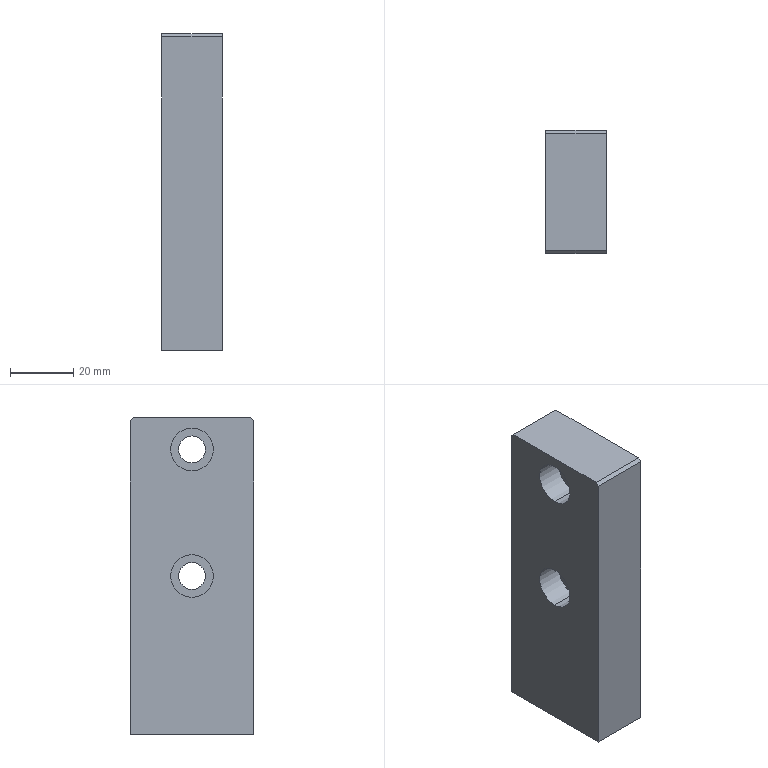Component | SolidWorks | TAR-02-017RightSupportPlate-1 | 1 solid | 26 faces | box 19 x 39 x 100 mm | volume 68972 mm3 | cylinder 12 | plane 10 | cone 4 | commonest cylinder face diameters 6.8 x4 13.5 x4 8.5 x4
build123d program:
from build123d import *

# Parameters (mm, degrees)
SKETCH1_W                                            = 100
SKETCH1_H                                            = 39
BOSS_EXTRUDE1_DEPTH                                  = 19
CYLINDRICAL_COUNTERSUNK_HOLE_FOR_M6_HEX_D            = 8.5
CYLINDRICAL_COUNTERSUNK_HOLE_FOR_M6_HEX_CBORE_D      = 13.5
CYLINDRICAL_COUNTERSUNK_HOLE_FOR_M6_HEX_CBORE_DEPTH  = 8.5
M6_HEX_HEAD_BOLT_CYLINDRICAL_COUNTERSUNK_D           = 8.5
M6_HEX_HEAD_BOLT_CYLINDRICAL_COUNTERSUNK_CBORE_D     = 13.5
M6_HEX_HEAD_BOLT_CYLINDRICAL_COUNTERSUNK_CBORE_DEPTH = 8.5
CHAMFER1_SIZE                                        = 1
M8_TAPPED_HOLE1_D                                    = 6.8
M8_TAPPED_HOLE1_DEPTH                                = 19.75
M8_TAPPED_HOLE1_TIP                                  = 2.043


with BuildPart() as part:
    # Sketch1 → Boss-Extrude1 (new body)
    with BuildSketch(Plane(origin=(0, 0, 0), x_dir=(0, 0, -1), z_dir=(1, 0, 0))):
        Rectangle(SKETCH1_W, SKETCH1_H)
    extrude(amount=BOSS_EXTRUDE1_DEPTH)

    # Cylindrical Countersunk Hole for M6 Hex (through all)
    with Locations(Plane(origin=(19, 0, 40), x_dir=(0, 0, 1), z_dir=(1, 0, 0))):
        with Locations((0, 0)):
            CounterBoreHole(CYLINDRICAL_COUNTERSUNK_HOLE_FOR_M6_HEX_D / 2, CYLINDRICAL_COUNTERSUNK_HOLE_FOR_M6_HEX_CBORE_D / 2, CYLINDRICAL_COUNTERSUNK_HOLE_FOR_M6_HEX_CBORE_DEPTH)

    # M6 Hex Head Bolt Cylindrical Countersunk (through all)
    with Locations(Plane(origin=(19, 0, 0), x_dir=(0, 0, 1), z_dir=(1, 0, 0))):
        with Locations((0, 0)):
            CounterBoreHole(M6_HEX_HEAD_BOLT_CYLINDRICAL_COUNTERSUNK_D / 2, M6_HEX_HEAD_BOLT_CYLINDRICAL_COUNTERSUNK_CBORE_D / 2, M6_HEX_HEAD_BOLT_CYLINDRICAL_COUNTERSUNK_CBORE_DEPTH)

    # Chamfer1
    chamfer1_edges = [part.edges().sort_by_distance(p)[0] for p in [
        (9.5, 19.5, 50),
        (9.5, -19.5, 50),
    ]]
    chamfer(chamfer1_edges, length=CHAMFER1_SIZE)

    # M8 Tapped Hole1
    with Locations(Plane(origin=(9.5, 10, -50), x_dir=(-1, 0, 0), z_dir=(0, 0, -1))):
        with Locations((0, 0), (0, -20)):
            Hole(M8_TAPPED_HOLE1_D / 2, depth=M8_TAPPED_HOLE1_DEPTH)
            with Locations((0, 0, -(M8_TAPPED_HOLE1_DEPTH + M8_TAPPED_HOLE1_TIP / 2))):  # 118° drill point
                Cone(0, M8_TAPPED_HOLE1_D / 2, M8_TAPPED_HOLE1_TIP, mode=Mode.SUBTRACT)


solid = part.part

# Placed as in the assembly
solid = solid.moved(Location((-44.891, 9.288, 59.5), (0, 0, 180)))
STEP:
#1=COLOUR_RGB('',0.7922,0.8196,0.9333);
#2=FILL_AREA_STYLE_COLOUR('',#1);
#3=FILL_AREA_STYLE('',(#2));
#4=SURFACE_STYLE_FILL_AREA(#3);
#5=SURFACE_SIDE_STYLE('',(#4));
#6=SURFACE_STYLE_USAGE(.BOTH.,#5);
#7=PRESENTATION_STYLE_ASSIGNMENT((#6));
#8=CARTESIAN_POINT('',(-2.275,-0.02804,1.152));
#9=VERTEX_POINT('',#8);
#10=CARTESIAN_POINT('',(-2.008,-0.02804,1.152));
#11=VERTEX_POINT('',#10);
#12=CARTESIAN_POINT('',(-2.141,-0.02804,1.152));
#13=DIRECTION('',(0.,0.,-1.));
#14=DIRECTION('',(1.,-0.,0.));
#15=AXIS2_PLACEMENT_3D('',#12,#13,#14);
#16=CIRCLE('',#15,0.1339);
#17=EDGE_CURVE('',#9,#11,#16,.T.);
#18=ORIENTED_EDGE('',*,*,#17,.F.);
#19=CARTESIAN_POINT('',(-2.275,-0.02804,0.374));
#20=VERTEX_POINT('',#19);
#21=CARTESIAN_POINT('',(-2.275,-0.02804,0.374));
#22=DIRECTION('',(0.,0.,-1.));
#23=VECTOR('',#22,39.37);
#24=LINE('',#21,#23);
#25=EDGE_CURVE('',#9,#20,#24,.T.);
#26=ORIENTED_EDGE('',*,*,#25,.T.);
#27=CARTESIAN_POINT('',(-2.008,-0.02804,0.374));
#28=VERTEX_POINT('',#27);
#29=CARTESIAN_POINT('',(-2.141,-0.02804,0.374));
#30=DIRECTION('',(0.,0.,-1.));
#31=DIRECTION('',(1.,-0.,0.));
#32=AXIS2_PLACEMENT_3D('',#29,#30,#31);
#33=CIRCLE('',#32,0.1339);
#34=EDGE_CURVE('',#20,#28,#33,.T.);
#35=ORIENTED_EDGE('',*,*,#34,.T.);
#36=CARTESIAN_POINT('',(-2.008,-0.02804,0.374));
#37=DIRECTION('',(0.,0.,-1.));
#38=VECTOR('',#37,39.37);
#39=LINE('',#36,#38);
#40=EDGE_CURVE('',#11,#28,#39,.T.);
#41=ORIENTED_EDGE('',*,*,#40,.F.);
#42=EDGE_LOOP('',(#18,#26,#35,#41));
#43=FACE_OUTER_BOUND('',#42,.T.);
#44=CARTESIAN_POINT('',(-2.141,-0.02804,0.374));
#45=DIRECTION('',(0.,0.,-1.));
#46=DIRECTION('',(1.,-0.,0.));
#47=AXIS2_PLACEMENT_3D('',#44,#45,#46);
#48=CYLINDRICAL_SURFACE('',#47,0.1339);
#49=ADVANCED_FACE('',(#43),#48,.F.);
#50=CARTESIAN_POINT('',(-2.141,-0.02804,1.232));
#51=VERTEX_POINT('',#50);
#52=CARTESIAN_POINT('',(-2.008,-0.02804,1.152));
#53=DIRECTION('',(0.8572,-0.,-0.515));
#54=VECTOR('',#53,39.37);
#55=LINE('',#52,#54);
#56=EDGE_CURVE('',#51,#11,#55,.T.);
#57=ORIENTED_EDGE('',*,*,#56,.F.);
#58=CARTESIAN_POINT('',(-2.275,-0.02804,1.152));
#59=DIRECTION('',(-0.8572,0.,-0.515));
#60=VECTOR('',#59,39.37);
#61=LINE('',#58,#60);
#62=EDGE_CURVE('',#51,#9,#61,.T.);
#63=ORIENTED_EDGE('',*,*,#62,.T.);
#64=ORIENTED_EDGE('',*,*,#17,.T.);
#65=EDGE_LOOP('',(#57,#63,#64));
#66=FACE_OUTER_BOUND('',#65,.T.);
#67=CARTESIAN_POINT('',(-2.141,-0.02804,1.152));
#68=DIRECTION('',(0.,0.,-1.));
#69=DIRECTION('',(1.,-0.,0.));
#70=AXIS2_PLACEMENT_3D('',#67,#68,#69);
#71=CONICAL_SURFACE('',#70,0.1339,1.03);
#72=ADVANCED_FACE('',(#66),#71,.F.);
#73=CARTESIAN_POINT('',(-2.275,0.7594,1.152));
#74=VERTEX_POINT('',#73);
#75=CARTESIAN_POINT('',(-2.008,0.7594,1.152));
#76=VERTEX_POINT('',#75);
#77=CARTESIAN_POINT('',(-2.141,0.7594,1.152));
#78=DIRECTION('',(0.,0.,-1.));
#79=DIRECTION('',(1.,0.,0.));
#80=AXIS2_PLACEMENT_3D('',#77,#78,#79);
#81=CIRCLE('',#80,0.1339);
#82=EDGE_CURVE('',#74,#76,#81,.T.);
#83=ORIENTED_EDGE('',*,*,#82,.F.);
#84=CARTESIAN_POINT('',(-2.275,0.7594,0.374));
#85=VERTEX_POINT('',#84);
#86=CARTESIAN_POINT('',(-2.275,0.7594,0.374));
#87=DIRECTION('',(0.,0.,-1.));
#88=VECTOR('',#87,39.37);
#89=LINE('',#86,#88);
#90=EDGE_CURVE('',#74,#85,#89,.T.);
#91=ORIENTED_EDGE('',*,*,#90,.T.);
#92=CARTESIAN_POINT('',(-2.008,0.7594,0.374));
#93=VERTEX_POINT('',#92);
#94=CARTESIAN_POINT('',(-2.141,0.7594,0.374));
#95=DIRECTION('',(0.,0.,-1.));
#96=DIRECTION('',(1.,0.,0.));
#97=AXIS2_PLACEMENT_3D('',#94,#95,#96);
#98=CIRCLE('',#97,0.1339);
#99=EDGE_CURVE('',#85,#93,#98,.T.);
#100=ORIENTED_EDGE('',*,*,#99,.T.);
#101=CARTESIAN_POINT('',(-2.008,0.7594,0.374));
#102=DIRECTION('',(0.,0.,-1.));
#103=VECTOR('',#102,39.37);
#104=LINE('',#101,#103);
#105=EDGE_CURVE('',#76,#93,#104,.T.);
#106=ORIENTED_EDGE('',*,*,#105,.F.);
#107=EDGE_LOOP('',(#83,#91,#100,#106));
#108=FACE_OUTER_BOUND('',#107,.T.);
#109=CARTESIAN_POINT('',(-2.141,0.7594,0.374));
#110=DIRECTION('',(0.,0.,-1.));
#111=DIRECTION('',(1.,0.,0.));
#112=AXIS2_PLACEMENT_3D('',#109,#110,#111);
#113=CYLINDRICAL_SURFACE('',#112,0.1339);
#114=ADVANCED_FACE('',(#108),#113,.F.);
#115=CARTESIAN_POINT('',(-2.141,0.7594,1.232));
#116=VERTEX_POINT('',#115);
#117=CARTESIAN_POINT('',(-2.008,0.7594,1.152));
#118=DIRECTION('',(0.8572,-0.,-0.515));
#119=VECTOR('',#118,39.37);
#120=LINE('',#117,#119);
#121=EDGE_CURVE('',#116,#76,#120,.T.);
#122=ORIENTED_EDGE('',*,*,#121,.F.);
#123=CARTESIAN_POINT('',(-2.275,0.7594,1.152));
#124=DIRECTION('',(-0.8572,0.,-0.515));
#125=VECTOR('',#124,39.37);
#126=LINE('',#123,#125);
#127=EDGE_CURVE('',#116,#74,#126,.T.);
#128=ORIENTED_EDGE('',*,*,#127,.T.);
#129=ORIENTED_EDGE('',*,*,#82,.T.);
#130=EDGE_LOOP('',(#122,#128,#129));
#131=FACE_OUTER_BOUND('',#130,.T.);
#132=CARTESIAN_POINT('',(-2.141,0.7594,1.152));
#133=DIRECTION('',(0.,0.,-1.));
#134=DIRECTION('',(1.,0.,0.));
#135=AXIS2_PLACEMENT_3D('',#132,#133,#134);
#136=CONICAL_SURFACE('',#135,0.1339,1.03);
#137=ADVANCED_FACE('',(#131),#136,.F.);
#138=CARTESIAN_POINT('',(-2.181,0.3657,2.608));
#139=VERTEX_POINT('',#138);
#140=CARTESIAN_POINT('',(-2.181,0.3657,2.077));
#141=VERTEX_POINT('',#140);
#142=CARTESIAN_POINT('',(-2.181,0.3657,2.343));
#143=DIRECTION('',(-1.,0.,0.));
#144=DIRECTION('',(0.,0.,-1.));
#145=AXIS2_PLACEMENT_3D('',#142,#143,#144);
#146=CIRCLE('',#145,0.2657);
#147=EDGE_CURVE('',#139,#141,#146,.T.);
#148=ORIENTED_EDGE('',*,*,#147,.F.);
#149=CARTESIAN_POINT('',(-2.515,0.3657,2.608));
#150=VERTEX_POINT('',#149);
#151=CARTESIAN_POINT('',(-2.515,0.3657,2.608));
#152=DIRECTION('',(-1.,0.,0.));
#153=VECTOR('',#152,39.37);
#154=LINE('',#151,#153);
#155=EDGE_CURVE('',#139,#150,#154,.T.);
#156=ORIENTED_EDGE('',*,*,#155,.T.);
#157=CARTESIAN_POINT('',(-2.515,0.3657,2.077));
#158=VERTEX_POINT('',#157);
#159=CARTESIAN_POINT('',(-2.515,0.3657,2.343));
#160=DIRECTION('',(-1.,0.,0.));
#161=DIRECTION('',(0.,0.,-1.));
#162=AXIS2_PLACEMENT_3D('',#159,#160,#161);
#163=CIRCLE('',#162,0.2657);
#164=EDGE_CURVE('',#150,#158,#163,.T.);
#165=ORIENTED_EDGE('',*,*,#164,.T.);
#166=CARTESIAN_POINT('',(-2.515,0.3657,2.077));
#167=DIRECTION('',(-1.,0.,0.));
#168=VECTOR('',#167,39.37);
#169=LINE('',#166,#168);
#170=EDGE_CURVE('',#141,#158,#169,.T.);
#171=ORIENTED_EDGE('',*,*,#170,.F.);
#172=EDGE_LOOP('',(#148,#156,#165,#171));
#173=FACE_OUTER_BOUND('',#172,.T.);
#174=CARTESIAN_POINT('',(-2.515,0.3657,2.343));
#175=DIRECTION('',(-1.,0.,0.));
#176=DIRECTION('',(0.,0.,-1.));
#177=AXIS2_PLACEMENT_3D('',#174,#175,#176);
#178=CYLINDRICAL_SURFACE('',#177,0.2657);
#179=ADVANCED_FACE('',(#173),#178,.F.);
#180=CARTESIAN_POINT('',(-1.767,0.3657,2.51));
#181=VERTEX_POINT('',#180);
#182=CARTESIAN_POINT('',(-1.767,0.3657,2.175));
#183=VERTEX_POINT('',#182);
#184=CARTESIAN_POINT('',(-1.767,0.3657,2.343));
#185=DIRECTION('',(-1.,0.,0.));
#186=DIRECTION('',(0.,0.,-1.));
#187=AXIS2_PLACEMENT_3D('',#184,#185,#186);
#188=CIRCLE('',#187,0.1673);
#189=EDGE_CURVE('',#181,#183,#188,.T.);
#190=ORIENTED_EDGE('',*,*,#189,.F.);
#191=CARTESIAN_POINT('',(-2.181,0.3657,2.51));
#192=VERTEX_POINT('',#191);
#193=CARTESIAN_POINT('',(-2.515,0.3657,2.51));
#194=DIRECTION('',(-1.,0.,0.));
#195=VECTOR('',#194,39.37);
#196=LINE('',#193,#195);
#197=EDGE_CURVE('',#181,#192,#196,.T.);
#198=ORIENTED_EDGE('',*,*,#197,.T.);
#199=CARTESIAN_POINT('',(-2.181,0.3657,2.175));
#200=VERTEX_POINT('',#199);
#201=CARTESIAN_POINT('',(-2.181,0.3657,2.343));
#202=DIRECTION('',(-1.,0.,0.));
#203=DIRECTION('',(0.,0.,-1.));
#204=AXIS2_PLACEMENT_3D('',#201,#202,#203);
#205=CIRCLE('',#204,0.1673);
#206=EDGE_CURVE('',#192,#200,#205,.T.);
#207=ORIENTED_EDGE('',*,*,#206,.T.);
#208=CARTESIAN_POINT('',(-2.515,0.3657,2.175));
#209=DIRECTION('',(-1.,0.,0.));
#210=VECTOR('',#209,39.37);
#211=LINE('',#208,#210);
#212=EDGE_CURVE('',#183,#200,#211,.T.);
#213=ORIENTED_EDGE('',*,*,#212,.F.);
#214=EDGE_LOOP('',(#190,#198,#207,#213));
#215=FACE_OUTER_BOUND('',#214,.T.);
#216=CARTESIAN_POINT('',(-2.515,0.3657,2.343));
#217=DIRECTION('',(-1.,0.,0.));
#218=DIRECTION('',(0.,0.,-1.));
#219=AXIS2_PLACEMENT_3D('',#216,#217,#218);
#220=CYLINDRICAL_SURFACE('',#219,0.1673);
#221=ADVANCED_FACE('',(#215),#220,.F.);
#222=CARTESIAN_POINT('',(-2.181,0.3657,4.183));
#223=VERTEX_POINT('',#222);
#224=CARTESIAN_POINT('',(-2.181,0.3657,3.652));
#225=VERTEX_POINT('',#224);
#226=CARTESIAN_POINT('',(-2.181,0.3657,3.917));
#227=DIRECTION('',(-1.,0.,0.));
#228=DIRECTION('',(0.,0.,-1.));
#229=AXIS2_PLACEMENT_3D('',#226,#227,#228);
#230=CIRCLE('',#229,0.2657);
#231=EDGE_CURVE('',#223,#225,#230,.T.);
#232=ORIENTED_EDGE('',*,*,#231,.F.);
#233=CARTESIAN_POINT('',(-2.515,0.3657,4.183));
#234=VERTEX_POINT('',#233);
#235=CARTESIAN_POINT('',(-2.515,0.3657,4.183));
#236=DIRECTION('',(-1.,0.,0.));
#237=VECTOR('',#236,39.37);
#238=LINE('',#235,#237);
#239=EDGE_CURVE('',#223,#234,#238,.T.);
#240=ORIENTED_EDGE('',*,*,#239,.T.);
#241=CARTESIAN_POINT('',(-2.515,0.3657,3.652));
#242=VERTEX_POINT('',#241);
#243=CARTESIAN_POINT('',(-2.515,0.3657,3.917));
#244=DIRECTION('',(-1.,0.,0.));
#245=DIRECTION('',(0.,0.,-1.));
#246=AXIS2_PLACEMENT_3D('',#243,#244,#245);
#247=CIRCLE('',#246,0.2657);
#248=EDGE_CURVE('',#234,#242,#247,.T.);
#249=ORIENTED_EDGE('',*,*,#248,.T.);
#250=CARTESIAN_POINT('',(-2.515,0.3657,3.652));
#251=DIRECTION('',(-1.,0.,0.));
#252=VECTOR('',#251,39.37);
#253=LINE('',#250,#252);
#254=EDGE_CURVE('',#225,#242,#253,.T.);
#255=ORIENTED_EDGE('',*,*,#254,.F.);
#256=EDGE_LOOP('',(#232,#240,#249,#255));
#257=FACE_OUTER_BOUND('',#256,.T.);
#258=CARTESIAN_POINT('',(-2.515,0.3657,3.917));
#259=DIRECTION('',(-1.,0.,0.));
#260=DIRECTION('',(0.,0.,-1.));
#261=AXIS2_PLACEMENT_3D('',#258,#259,#260);
#262=CYLINDRICAL_SURFACE('',#261,0.2657);
#263=ADVANCED_FACE('',(#257),#262,.F.);
#264=CARTESIAN_POINT('',(-1.767,0.3657,4.085));
#265=VERTEX_POINT('',#264);
#266=CARTESIAN_POINT('',(-1.767,0.3657,3.75));
#267=VERTEX_POINT('',#266);
#268=CARTESIAN_POINT('',(-1.767,0.3657,3.917));
#269=DIRECTION('',(-1.,0.,0.));
#270=DIRECTION('',(0.,0.,-1.));
#271=AXIS2_PLACEMENT_3D('',#268,#269,#270);
#272=CIRCLE('',#271,0.1673);
#273=EDGE_CURVE('',#265,#267,#272,.T.);
#274=ORIENTED_EDGE('',*,*,#273,.F.);
#275=CARTESIAN_POINT('',(-2.181,0.3657,4.085));
#276=VERTEX_POINT('',#275);
#277=CARTESIAN_POINT('',(-2.515,0.3657,4.085));
#278=DIRECTION('',(-1.,0.,0.));
#279=VECTOR('',#278,39.37);
#280=LINE('',#277,#279);
#281=EDGE_CURVE('',#265,#276,#280,.T.);
#282=ORIENTED_EDGE('',*,*,#281,.T.);
#283=CARTESIAN_POINT('',(-2.181,0.3657,3.75));
#284=VERTEX_POINT('',#283);
#285=CARTESIAN_POINT('',(-2.181,0.3657,3.917));
#286=DIRECTION('',(-1.,0.,0.));
#287=DIRECTION('',(0.,0.,-1.));
#288=AXIS2_PLACEMENT_3D('',#285,#286,#287);
#289=CIRCLE('',#288,0.1673);
#290=EDGE_CURVE('',#276,#284,#289,.T.);
#291=ORIENTED_EDGE('',*,*,#290,.T.);
#292=CARTESIAN_POINT('',(-2.515,0.3657,3.75));
#293=DIRECTION('',(-1.,0.,0.));
#294=VECTOR('',#293,39.37);
#295=LINE('',#292,#294);
#296=EDGE_CURVE('',#267,#284,#295,.T.);
#297=ORIENTED_EDGE('',*,*,#296,.F.);
#298=EDGE_LOOP('',(#274,#282,#291,#297));
#299=FACE_OUTER_BOUND('',#298,.T.);
#300=CARTESIAN_POINT('',(-2.515,0.3657,3.917));
#301=DIRECTION('',(-1.,0.,0.));
#302=DIRECTION('',(0.,0.,-1.));
#303=AXIS2_PLACEMENT_3D('',#300,#301,#302);
#304=CYLINDRICAL_SURFACE('',#303,0.1673);
#305=ADVANCED_FACE('',(#299),#304,.F.);
#306=CARTESIAN_POINT('',(-1.767,-0.3627,4.311));
#307=VERTEX_POINT('',#306);
#308=CARTESIAN_POINT('',(-1.767,1.094,4.311));
#309=VERTEX_POINT('',#308);
#310=CARTESIAN_POINT('',(-1.767,1.133,4.311));
#311=DIRECTION('',(0.,1.,0.));
#312=VECTOR('',#311,39.37);
#313=LINE('',#310,#312);
#314=EDGE_CURVE('',#307,#309,#313,.T.);
#315=ORIENTED_EDGE('',*,*,#314,.T.);
#316=CARTESIAN_POINT('',(-2.515,1.094,4.311));
#317=VERTEX_POINT('',#316);
#318=CARTESIAN_POINT('',(-2.515,1.094,4.311));
#319=DIRECTION('',(-1.,0.,0.));
#320=VECTOR('',#319,39.37);
#321=LINE('',#318,#320);
#322=EDGE_CURVE('',#309,#317,#321,.T.);
#323=ORIENTED_EDGE('',*,*,#322,.T.);
#324=CARTESIAN_POINT('',(-2.515,-0.3627,4.311));
#325=VERTEX_POINT('',#324);
#326=CARTESIAN_POINT('',(-2.515,1.133,4.311));
#327=DIRECTION('',(0.,1.,0.));
#328=VECTOR('',#327,39.37);
#329=LINE('',#326,#328);
#330=EDGE_CURVE('',#325,#317,#329,.T.);
#331=ORIENTED_EDGE('',*,*,#330,.F.);
#332=CARTESIAN_POINT('',(-2.515,-0.3627,4.311));
#333=DIRECTION('',(1.,-0.,0.));
#334=VECTOR('',#333,39.37);
#335=LINE('',#332,#334);
#336=EDGE_CURVE('',#325,#307,#335,.T.);
#337=ORIENTED_EDGE('',*,*,#336,.T.);
#338=EDGE_LOOP('',(#315,#323,#331,#337));
#339=FACE_OUTER_BOUND('',#338,.T.);
#340=CARTESIAN_POINT('',(-2.515,1.133,4.311));
#341=DIRECTION('',(0.,0.,-1.));
#342=DIRECTION('',(1.,-0.,0.));
#343=AXIS2_PLACEMENT_3D('',#340,#341,#342);
#344=PLANE('',#343);
#345=ADVANCED_FACE('',(#339),#344,.F.);
#346=CARTESIAN_POINT('',(-2.515,1.133,4.272));
#347=VERTEX_POINT('',#346);
#348=CARTESIAN_POINT('',(-2.515,1.133,0.374));
#349=VERTEX_POINT('',#348);
#350=CARTESIAN_POINT('',(-2.515,1.133,0.374));
#351=DIRECTION('',(-0.,-0.,-1.));
#352=VECTOR('',#351,39.37);
#353=LINE('',#350,#352);
#354=EDGE_CURVE('',#347,#349,#353,.T.);
#355=ORIENTED_EDGE('',*,*,#354,.F.);
#356=CARTESIAN_POINT('',(-1.767,1.133,4.272));
#357=VERTEX_POINT('',#356);
#358=CARTESIAN_POINT('',(-2.515,1.133,4.272));
#359=DIRECTION('',(1.,-0.,0.));
#360=VECTOR('',#359,39.37);
#361=LINE('',#358,#360);
#362=EDGE_CURVE('',#347,#357,#361,.T.);
#363=ORIENTED_EDGE('',*,*,#362,.T.);
#364=CARTESIAN_POINT('',(-1.767,1.133,0.374));
#365=VERTEX_POINT('',#364);
#366=CARTESIAN_POINT('',(-1.767,1.133,0.374));
#367=DIRECTION('',(-0.,-0.,-1.));
#368=VECTOR('',#367,39.37);
#369=LINE('',#366,#368);
#370=EDGE_CURVE('',#357,#365,#369,.T.);
#371=ORIENTED_EDGE('',*,*,#370,.T.);
#372=CARTESIAN_POINT('',(-2.515,1.133,0.374));
#373=DIRECTION('',(1.,-0.,0.));
#374=VECTOR('',#373,39.37);
#375=LINE('',#372,#374);
#376=EDGE_CURVE('',#349,#365,#375,.T.);
#377=ORIENTED_EDGE('',*,*,#376,.F.);
#378=EDGE_LOOP('',(#355,#363,#371,#377));
#379=FACE_OUTER_BOUND('',#378,.T.);
#380=CARTESIAN_POINT('',(-2.515,1.133,0.374));
#381=DIRECTION('',(-0.,-1.,0.));
#382=DIRECTION('',(0.,0.,1.));
#383=AXIS2_PLACEMENT_3D('',#380,#381,#382);
#384=PLANE('',#383);
#385=ADVANCED_FACE('',(#379),#384,.F.);
#386=CARTESIAN_POINT('',(-2.141,-0.02804,0.374));
#387=DIRECTION('',(0.,0.,-1.));
#388=DIRECTION('',(1.,-0.,0.));
#389=AXIS2_PLACEMENT_3D('',#386,#387,#388);
#390=CIRCLE('',#389,0.1339);
#391=EDGE_CURVE('',#28,#20,#390,.T.);
#392=ORIENTED_EDGE('',*,*,#391,.F.);
#393=ORIENTED_EDGE('',*,*,#34,.F.);
#394=EDGE_LOOP('',(#392,#393));
#395=FACE_BOUND('',#394,.T.);
#396=CARTESIAN_POINT('',(-2.141,0.7594,0.374));
#397=DIRECTION('',(0.,0.,-1.));
#398=DIRECTION('',(1.,0.,0.));
#399=AXIS2_PLACEMENT_3D('',#396,#397,#398);
#400=CIRCLE('',#399,0.1339);
#401=EDGE_CURVE('',#93,#85,#400,.T.);
#402=ORIENTED_EDGE('',*,*,#401,.F.);
#403=ORIENTED_EDGE('',*,*,#99,.F.);
#404=EDGE_LOOP('',(#402,#403));
#405=FACE_BOUND('',#404,.T.);
#406=CARTESIAN_POINT('',(-1.767,-0.4021,0.374));
#407=VERTEX_POINT('',#406);
#408=CARTESIAN_POINT('',(-1.767,1.133,0.374));
#409=DIRECTION('',(-0.,-1.,0.));
#410=VECTOR('',#409,39.37);
#411=LINE('',#408,#410);
#412=EDGE_CURVE('',#365,#407,#411,.T.);
#413=ORIENTED_EDGE('',*,*,#412,.T.);
#414=CARTESIAN_POINT('',(-2.515,-0.4021,0.374));
#415=VERTEX_POINT('',#414);
#416=CARTESIAN_POINT('',(-2.515,-0.4021,0.374));
#417=DIRECTION('',(1.,-0.,0.));
#418=VECTOR('',#417,39.37);
#419=LINE('',#416,#418);
#420=EDGE_CURVE('',#415,#407,#419,.T.);
#421=ORIENTED_EDGE('',*,*,#420,.F.);
#422=CARTESIAN_POINT('',(-2.515,1.133,0.374));
#423=DIRECTION('',(-0.,-1.,0.));
#424=VECTOR('',#423,39.37);
#425=LINE('',#422,#424);
#426=EDGE_CURVE('',#349,#415,#425,.T.);
#427=ORIENTED_EDGE('',*,*,#426,.F.);
#428=ORIENTED_EDGE('',*,*,#376,.T.);
#429=EDGE_LOOP('',(#413,#421,#427,#428));
#430=FACE_OUTER_BOUND('',#429,.T.);
#431=CARTESIAN_POINT('',(-2.515,1.133,0.374));
#432=DIRECTION('',(0.,0.,1.));
#433=DIRECTION('',(-1.,0.,0.));
#434=AXIS2_PLACEMENT_3D('',#431,#432,#433);
#435=PLANE('',#434);
#436=ADVANCED_FACE('',(#395,#405,#430),#435,.F.);
#437=CARTESIAN_POINT('',(-1.767,-0.4021,4.272));
#438=VERTEX_POINT('',#437);
#439=CARTESIAN_POINT('',(-1.767,-0.4021,0.374));
#440=DIRECTION('',(0.,0.,1.));
#441=VECTOR('',#440,39.37);
#442=LINE('',#439,#441);
#443=EDGE_CURVE('',#407,#438,#442,.T.);
#444=ORIENTED_EDGE('',*,*,#443,.T.);
#445=CARTESIAN_POINT('',(-2.515,-0.4021,4.272));
#446=VERTEX_POINT('',#445);
#447=CARTESIAN_POINT('',(-2.515,-0.4021,4.272));
#448=DIRECTION('',(-1.,0.,0.));
#449=VECTOR('',#448,39.37);
#450=LINE('',#447,#449);
#451=EDGE_CURVE('',#438,#446,#450,.T.);
#452=ORIENTED_EDGE('',*,*,#451,.T.);
#453=CARTESIAN_POINT('',(-2.515,-0.4021,0.374));
#454=DIRECTION('',(0.,0.,1.));
#455=VECTOR('',#454,39.37);
#456=LINE('',#453,#455);
#457=EDGE_CURVE('',#415,#446,#456,.T.);
#458=ORIENTED_EDGE('',*,*,#457,.F.);
#459=ORIENTED_EDGE('',*,*,#420,.T.);
#460=EDGE_LOOP('',(#444,#452,#458,#459));
#461=FACE_OUTER_BOUND('',#460,.T.);
#462=CARTESIAN_POINT('',(-2.515,-0.4021,0.374));
#463=DIRECTION('',(0.,1.,-0.));
#464=DIRECTION('',(-0.,-0.,-1.));
#465=AXIS2_PLACEMENT_3D('',#462,#463,#464);
#466=PLANE('',#465);
#467=ADVANCED_FACE('',(#461),#466,.F.);
#468=CARTESIAN_POINT('',(-2.515,0.3657,2.343));
#469=DIRECTION('',(-1.,0.,0.));
#470=DIRECTION('',(0.,0.,-1.));
#471=AXIS2_PLACEMENT_3D('',#468,#469,#470);
#472=CIRCLE('',#471,0.2657);
#473=EDGE_CURVE('',#158,#150,#472,.T.);
#474=ORIENTED_EDGE('',*,*,#473,.F.);
#475=ORIENTED_EDGE('',*,*,#164,.F.);
#476=EDGE_LOOP('',(#474,#475));
#477=FACE_BOUND('',#476,.T.);
#478=CARTESIAN_POINT('',(-2.515,0.3657,3.917));
#479=DIRECTION('',(-1.,0.,0.));
#480=DIRECTION('',(0.,0.,-1.));
#481=AXIS2_PLACEMENT_3D('',#478,#479,#480);
#482=CIRCLE('',#481,0.2657);
#483=EDGE_CURVE('',#242,#234,#482,.T.);
#484=ORIENTED_EDGE('',*,*,#483,.F.);
#485=ORIENTED_EDGE('',*,*,#248,.F.);
#486=EDGE_LOOP('',(#484,#485));
#487=FACE_BOUND('',#486,.T.);
#488=ORIENTED_EDGE('',*,*,#330,.T.);
#489=CARTESIAN_POINT('',(-2.515,1.714,3.691));
#490=DIRECTION('',(0.,0.7071,-0.7071));
#491=VECTOR('',#490,39.37);
#492=LINE('',#489,#491);
#493=EDGE_CURVE('',#317,#347,#492,.T.);
#494=ORIENTED_EDGE('',*,*,#493,.T.);
#495=ORIENTED_EDGE('',*,*,#354,.T.);
#496=ORIENTED_EDGE('',*,*,#426,.T.);
#497=ORIENTED_EDGE('',*,*,#457,.T.);
#498=CARTESIAN_POINT('',(-2.515,-0.9828,3.691));
#499=DIRECTION('',(0.,0.7071,0.7071));
#500=VECTOR('',#499,39.37);
#501=LINE('',#498,#500);
#502=EDGE_CURVE('',#446,#325,#501,.T.);
#503=ORIENTED_EDGE('',*,*,#502,.T.);
#504=EDGE_LOOP('',(#488,#494,#495,#496,#497,#503));
#505=FACE_OUTER_BOUND('',#504,.T.);
#506=CARTESIAN_POINT('',(-2.515,0.3657,2.343));
#507=DIRECTION('',(-1.,0.,0.));
#508=DIRECTION('',(0.,0.,-1.));
#509=AXIS2_PLACEMENT_3D('',#506,#507,#508);
#510=PLANE('',#509);
#511=ADVANCED_FACE('',(#477,#487,#505),#510,.T.);
#512=CARTESIAN_POINT('',(-1.767,0.3657,2.343));
#513=DIRECTION('',(-1.,0.,0.));
#514=DIRECTION('',(0.,0.,-1.));
#515=AXIS2_PLACEMENT_3D('',#512,#513,#514);
#516=CIRCLE('',#515,0.1673);
#517=EDGE_CURVE('',#183,#181,#516,.T.);
#518=ORIENTED_EDGE('',*,*,#517,.T.);
#519=ORIENTED_EDGE('',*,*,#189,.T.);
#520=EDGE_LOOP('',(#518,#519));
#521=FACE_BOUND('',#520,.T.);
#522=CARTESIAN_POINT('',(-1.767,0.3657,3.917));
#523=DIRECTION('',(-1.,0.,0.));
#524=DIRECTION('',(0.,0.,-1.));
#525=AXIS2_PLACEMENT_3D('',#522,#523,#524);
#526=CIRCLE('',#525,0.1673);
#527=EDGE_CURVE('',#267,#265,#526,.T.);
#528=ORIENTED_EDGE('',*,*,#527,.T.);
#529=ORIENTED_EDGE('',*,*,#273,.T.);
#530=EDGE_LOOP('',(#528,#529));
#531=FACE_BOUND('',#530,.T.);
#532=ORIENTED_EDGE('',*,*,#370,.F.);
#533=CARTESIAN_POINT('',(-1.767,1.133,4.272));
#534=DIRECTION('',(-0.,-0.7071,0.7071));
#535=VECTOR('',#534,39.37);
#536=LINE('',#533,#535);
#537=EDGE_CURVE('',#357,#309,#536,.T.);
#538=ORIENTED_EDGE('',*,*,#537,.T.);
#539=ORIENTED_EDGE('',*,*,#314,.F.);
#540=CARTESIAN_POINT('',(-1.767,-0.3627,4.311));
#541=DIRECTION('',(-0.,-0.7071,-0.7071));
#542=VECTOR('',#541,39.37);
#543=LINE('',#540,#542);
#544=EDGE_CURVE('',#307,#438,#543,.T.);
#545=ORIENTED_EDGE('',*,*,#544,.T.);
#546=ORIENTED_EDGE('',*,*,#443,.F.);
#547=ORIENTED_EDGE('',*,*,#412,.F.);
#548=EDGE_LOOP('',(#532,#538,#539,#545,#546,#547));
#549=FACE_OUTER_BOUND('',#548,.T.);
#550=CARTESIAN_POINT('',(-1.767,0.3657,2.343));
#551=DIRECTION('',(-1.,0.,0.));
#552=DIRECTION('',(0.,0.,-1.));
#553=AXIS2_PLACEMENT_3D('',#550,#551,#552);
#554=PLANE('',#553);
#555=ADVANCED_FACE('',(#521,#531,#549),#554,.F.);
#556=ORIENTED_EDGE('',*,*,#281,.F.);
#557=ORIENTED_EDGE('',*,*,#527,.F.);
#558=ORIENTED_EDGE('',*,*,#296,.T.);
#559=CARTESIAN_POINT('',(-2.181,0.3657,3.917));
#560=DIRECTION('',(-1.,0.,0.));
#561=DIRECTION('',(0.,0.,-1.));
#562=AXIS2_PLACEMENT_3D('',#559,#560,#561);
#563=CIRCLE('',#562,0.1673);
#564=EDGE_CURVE('',#284,#276,#563,.T.);
#565=ORIENTED_EDGE('',*,*,#564,.T.);
#566=EDGE_LOOP('',(#556,#557,#558,#565));
#567=FACE_OUTER_BOUND('',#566,.T.);
#568=CARTESIAN_POINT('',(-2.515,0.3657,3.917));
#569=DIRECTION('',(-1.,0.,0.));
#570=DIRECTION('',(0.,0.,-1.));
#571=AXIS2_PLACEMENT_3D('',#568,#569,#570);
#572=CYLINDRICAL_SURFACE('',#571,0.1673);
#573=ADVANCED_FACE('',(#567),#572,.F.);
#574=ORIENTED_EDGE('',*,*,#564,.F.);
#575=ORIENTED_EDGE('',*,*,#290,.F.);
#576=EDGE_LOOP('',(#574,#575));
#577=FACE_BOUND('',#576,.T.);
#578=CARTESIAN_POINT('',(-2.181,0.3657,3.917));
#579=DIRECTION('',(-1.,0.,0.));
#580=DIRECTION('',(0.,0.,-1.));
#581=AXIS2_PLACEMENT_3D('',#578,#579,#580);
#582=CIRCLE('',#581,0.2657);
#583=EDGE_CURVE('',#225,#223,#582,.T.);
#584=ORIENTED_EDGE('',*,*,#583,.T.);
#585=ORIENTED_EDGE('',*,*,#231,.T.);
#586=EDGE_LOOP('',(#584,#585));
#587=FACE_OUTER_BOUND('',#586,.T.);
#588=CARTESIAN_POINT('',(-2.181,0.1983,3.917));
#589=DIRECTION('',(1.,-0.,0.));
#590=DIRECTION('',(0.,0.,1.));
#591=AXIS2_PLACEMENT_3D('',#588,#589,#590);
#592=PLANE('',#591);
#593=ADVANCED_FACE('',(#577,#587),#592,.F.);
#594=ORIENTED_EDGE('',*,*,#239,.F.);
#595=ORIENTED_EDGE('',*,*,#583,.F.);
#596=ORIENTED_EDGE('',*,*,#254,.T.);
#597=ORIENTED_EDGE('',*,*,#483,.T.);
#598=EDGE_LOOP('',(#594,#595,#596,#597));
#599=FACE_OUTER_BOUND('',#598,.T.);
#600=CARTESIAN_POINT('',(-2.515,0.3657,3.917));
#601=DIRECTION('',(-1.,0.,0.));
#602=DIRECTION('',(0.,0.,-1.));
#603=AXIS2_PLACEMENT_3D('',#600,#601,#602);
#604=CYLINDRICAL_SURFACE('',#603,0.2657);
#605=ADVANCED_FACE('',(#599),#604,.F.);
#606=ORIENTED_EDGE('',*,*,#197,.F.);
#607=ORIENTED_EDGE('',*,*,#517,.F.);
#608=ORIENTED_EDGE('',*,*,#212,.T.);
#609=CARTESIAN_POINT('',(-2.181,0.3657,2.343));
#610=DIRECTION('',(-1.,0.,0.));
#611=DIRECTION('',(0.,0.,-1.));
#612=AXIS2_PLACEMENT_3D('',#609,#610,#611);
#613=CIRCLE('',#612,0.1673);
#614=EDGE_CURVE('',#200,#192,#613,.T.);
#615=ORIENTED_EDGE('',*,*,#614,.T.);
#616=EDGE_LOOP('',(#606,#607,#608,#615));
#617=FACE_OUTER_BOUND('',#616,.T.);
#618=CARTESIAN_POINT('',(-2.515,0.3657,2.343));
#619=DIRECTION('',(-1.,0.,0.));
#620=DIRECTION('',(0.,0.,-1.));
#621=AXIS2_PLACEMENT_3D('',#618,#619,#620);
#622=CYLINDRICAL_SURFACE('',#621,0.1673);
#623=ADVANCED_FACE('',(#617),#622,.F.);
#624=ORIENTED_EDGE('',*,*,#614,.F.);
#625=ORIENTED_EDGE('',*,*,#206,.F.);
#626=EDGE_LOOP('',(#624,#625));
#627=FACE_BOUND('',#626,.T.);
#628=CARTESIAN_POINT('',(-2.181,0.3657,2.343));
#629=DIRECTION('',(-1.,0.,0.));
#630=DIRECTION('',(0.,0.,-1.));
#631=AXIS2_PLACEMENT_3D('',#628,#629,#630);
#632=CIRCLE('',#631,0.2657);
#633=EDGE_CURVE('',#141,#139,#632,.T.);
#634=ORIENTED_EDGE('',*,*,#633,.T.);
#635=ORIENTED_EDGE('',*,*,#147,.T.);
#636=EDGE_LOOP('',(#634,#635));
#637=FACE_OUTER_BOUND('',#636,.T.);
#638=CARTESIAN_POINT('',(-2.181,0.1983,2.343));
#639=DIRECTION('',(1.,-0.,0.));
#640=DIRECTION('',(0.,0.,1.));
#641=AXIS2_PLACEMENT_3D('',#638,#639,#640);
#642=PLANE('',#641);
#643=ADVANCED_FACE('',(#627,#637),#642,.F.);
#644=ORIENTED_EDGE('',*,*,#155,.F.);
#645=ORIENTED_EDGE('',*,*,#633,.F.);
#646=ORIENTED_EDGE('',*,*,#170,.T.);
#647=ORIENTED_EDGE('',*,*,#473,.T.);
#648=EDGE_LOOP('',(#644,#645,#646,#647));
#649=FACE_OUTER_BOUND('',#648,.T.);
#650=CARTESIAN_POINT('',(-2.515,0.3657,2.343));
#651=DIRECTION('',(-1.,0.,0.));
#652=DIRECTION('',(0.,0.,-1.));
#653=AXIS2_PLACEMENT_3D('',#650,#651,#652);
#654=CYLINDRICAL_SURFACE('',#653,0.2657);
#655=ADVANCED_FACE('',(#649),#654,.F.);
#656=ORIENTED_EDGE('',*,*,#493,.F.);
#657=ORIENTED_EDGE('',*,*,#322,.F.);
#658=ORIENTED_EDGE('',*,*,#537,.F.);
#659=ORIENTED_EDGE('',*,*,#362,.F.);
#660=EDGE_LOOP('',(#656,#657,#658,#659));
#661=FACE_OUTER_BOUND('',#660,.T.);
#662=CARTESIAN_POINT('',(-2.515,1.133,4.272));
#663=DIRECTION('',(-0.,-0.7071,-0.7071));
#664=DIRECTION('',(1.,-0.,0.));
#665=AXIS2_PLACEMENT_3D('',#662,#663,#664);
#666=PLANE('',#665);
#667=ADVANCED_FACE('',(#661),#666,.F.);
#668=ORIENTED_EDGE('',*,*,#502,.F.);
#669=ORIENTED_EDGE('',*,*,#451,.F.);
#670=ORIENTED_EDGE('',*,*,#544,.F.);
#671=ORIENTED_EDGE('',*,*,#336,.F.);
#672=EDGE_LOOP('',(#668,#669,#670,#671));
#673=FACE_OUTER_BOUND('',#672,.T.);
#674=CARTESIAN_POINT('',(-2.515,-0.3627,4.311));
#675=DIRECTION('',(0.,0.7071,-0.7071));
#676=DIRECTION('',(1.,-0.,0.));
#677=AXIS2_PLACEMENT_3D('',#674,#675,#676);
#678=PLANE('',#677);
#679=ADVANCED_FACE('',(#673),#678,.F.);
#680=ORIENTED_EDGE('',*,*,#127,.F.);
#681=ORIENTED_EDGE('',*,*,#121,.T.);
#682=CARTESIAN_POINT('',(-2.141,0.7594,1.152));
#683=DIRECTION('',(0.,0.,-1.));
#684=DIRECTION('',(1.,0.,0.));
#685=AXIS2_PLACEMENT_3D('',#682,#683,#684);
#686=CIRCLE('',#685,0.1339);
#687=EDGE_CURVE('',#76,#74,#686,.T.);
#688=ORIENTED_EDGE('',*,*,#687,.T.);
#689=EDGE_LOOP('',(#680,#681,#688));
#690=FACE_OUTER_BOUND('',#689,.T.);
#691=CARTESIAN_POINT('',(-2.141,0.7594,1.152));
#692=DIRECTION('',(0.,0.,-1.));
#693=DIRECTION('',(1.,0.,0.));
#694=AXIS2_PLACEMENT_3D('',#691,#692,#693);
#695=CONICAL_SURFACE('',#694,0.1339,1.03);
#696=ADVANCED_FACE('',(#690),#695,.F.);
#697=ORIENTED_EDGE('',*,*,#90,.F.);
#698=ORIENTED_EDGE('',*,*,#687,.F.);
#699=ORIENTED_EDGE('',*,*,#105,.T.);
#700=ORIENTED_EDGE('',*,*,#401,.T.);
#701=EDGE_LOOP('',(#697,#698,#699,#700));
#702=FACE_OUTER_BOUND('',#701,.T.);
#703=CARTESIAN_POINT('',(-2.141,0.7594,0.374));
#704=DIRECTION('',(0.,0.,-1.));
#705=DIRECTION('',(1.,0.,0.));
#706=AXIS2_PLACEMENT_3D('',#703,#704,#705);
#707=CYLINDRICAL_SURFACE('',#706,0.1339);
#708=ADVANCED_FACE('',(#702),#707,.F.);
#709=ORIENTED_EDGE('',*,*,#62,.F.);
#710=ORIENTED_EDGE('',*,*,#56,.T.);
#711=CARTESIAN_POINT('',(-2.141,-0.02804,1.152));
#712=DIRECTION('',(0.,0.,-1.));
#713=DIRECTION('',(1.,-0.,0.));
#714=AXIS2_PLACEMENT_3D('',#711,#712,#713);
#715=CIRCLE('',#714,0.1339);
#716=EDGE_CURVE('',#11,#9,#715,.T.);
#717=ORIENTED_EDGE('',*,*,#716,.T.);
#718=EDGE_LOOP('',(#709,#710,#717));
#719=FACE_OUTER_BOUND('',#718,.T.);
#720=CARTESIAN_POINT('',(-2.141,-0.02804,1.152));
#721=DIRECTION('',(0.,0.,-1.));
#722=DIRECTION('',(1.,-0.,0.));
#723=AXIS2_PLACEMENT_3D('',#720,#721,#722);
#724=CONICAL_SURFACE('',#723,0.1339,1.03);
#725=ADVANCED_FACE('',(#719),#724,.F.);
#726=ORIENTED_EDGE('',*,*,#25,.F.);
#727=ORIENTED_EDGE('',*,*,#716,.F.);
#728=ORIENTED_EDGE('',*,*,#40,.T.);
#729=ORIENTED_EDGE('',*,*,#391,.T.);
#730=EDGE_LOOP('',(#726,#727,#728,#729));
#731=FACE_OUTER_BOUND('',#730,.T.);
#732=CARTESIAN_POINT('',(-2.141,-0.02804,0.374));
#733=DIRECTION('',(0.,0.,-1.));
#734=DIRECTION('',(1.,-0.,0.));
#735=AXIS2_PLACEMENT_3D('',#732,#733,#734);
#736=CYLINDRICAL_SURFACE('',#735,0.1339);
#737=ADVANCED_FACE('',(#731),#736,.F.);
#738=CLOSED_SHELL('',(#49,#72,#114,#137,#179,#221,#263,#305,#345,#385,#436,#467,#511,#555,#573,#593,#605,#623,#643,#655,#667,#679,#696,#708,#725,#737));
#739=MANIFOLD_SOLID_BREP('',#738);
#740=STYLED_ITEM('',(#7),#739);
#741=PRESENTATION_LAYER_ASSIGNMENT('','',(#740));
#742=(LENGTH_UNIT()NAMED_UNIT(*)SI_UNIT($,.METRE.));
#743=LENGTH_MEASURE_WITH_UNIT(LENGTH_MEASURE(0.0254),#742);
#744=DIMENSIONAL_EXPONENTS(1.,0.,0.,0.,0.,0.,0.);
#745=(CONVERSION_BASED_UNIT('',#743)LENGTH_UNIT()NAMED_UNIT(#744));
#746=UNCERTAINTY_MEASURE_WITH_UNIT(LENGTH_MEASURE(0.00001),#745,'','');
#747=(NAMED_UNIT(*)PLANE_ANGLE_UNIT()SI_UNIT($,.RADIAN.));
#748=(NAMED_UNIT(*)SI_UNIT($,.STERADIAN.)SOLID_ANGLE_UNIT());
#749=(GEOMETRIC_REPRESENTATION_CONTEXT(3)GLOBAL_UNCERTAINTY_ASSIGNED_CONTEXT((#746))GLOBAL_UNIT_ASSIGNED_CONTEXT((#745,#747,#748))REPRESENTATION_CONTEXT('',''));
#750=MECHANICAL_DESIGN_GEOMETRIC_PRESENTATION_REPRESENTATION('',(#740),#749);
#751=CARTESIAN_POINT('',(0.,0.,0.));
#752=DIRECTION('',(0.,0.,1.));
#753=DIRECTION('',(1.,0.,0.));
#754=AXIS2_PLACEMENT_3D('',#751,#752,#753);
#755=(LENGTH_UNIT()NAMED_UNIT(*)SI_UNIT($,.METRE.));
#756=LENGTH_MEASURE_WITH_UNIT(LENGTH_MEASURE(0.0254),#755);
#757=DIMENSIONAL_EXPONENTS(1.,0.,0.,0.,0.,0.,0.);
#758=(CONVERSION_BASED_UNIT('',#756)LENGTH_UNIT()NAMED_UNIT(#757));
#759=UNCERTAINTY_MEASURE_WITH_UNIT(LENGTH_MEASURE(0.00001),#758,'','');
#760=(NAMED_UNIT(*)PLANE_ANGLE_UNIT()SI_UNIT($,.RADIAN.));
#761=(NAMED_UNIT(*)SI_UNIT($,.STERADIAN.)SOLID_ANGLE_UNIT());
#762=(GEOMETRIC_REPRESENTATION_CONTEXT(3)GLOBAL_UNCERTAINTY_ASSIGNED_CONTEXT((#759))GLOBAL_UNIT_ASSIGNED_CONTEXT((#758,#760,#761))REPRESENTATION_CONTEXT('',''));
#763=ADVANCED_BREP_SHAPE_REPRESENTATION('',(#739,#754),#762);